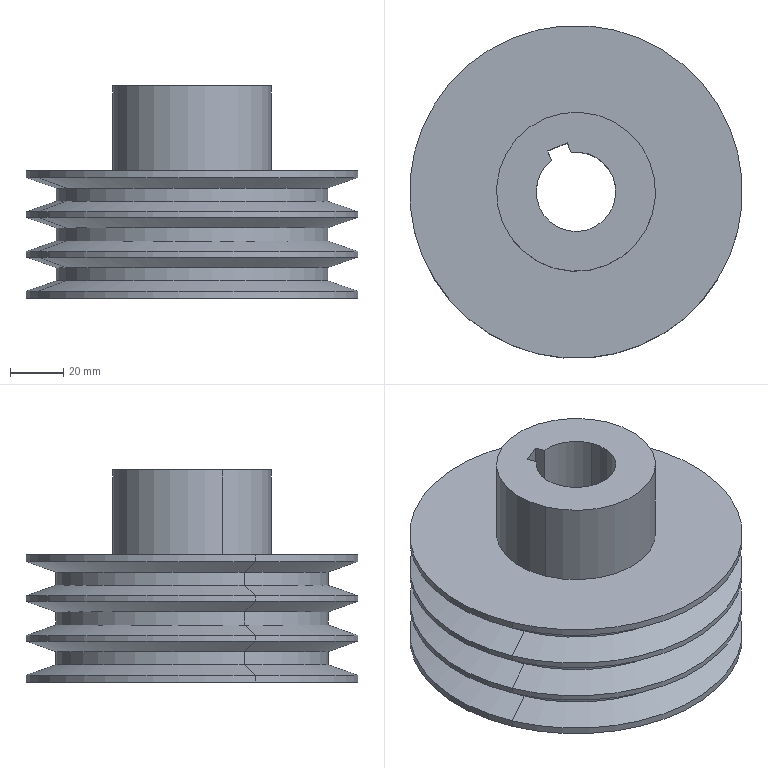Component | SolidWorks | SmallPulley-2 | 1 solid | 47 faces | box 125.5 x 125.5 x 80 mm | volume 513593 mm3 | cylinder 22 | cone 18 | plane 7 | commonest cylinder face diameters 125.5 x8 30 x6 102.6 x6 60 x2
build123d program:
from build123d import *

# Parameters (mm, degrees)
LPATTERN1_COUNT     = 3
LPATTERN1_PITCH     = 15
CHAMFER1_SIZE       = 1
SKETCH4_W           = 8
SKETCH4_H           = 3.843
CUT_EXTRUDE1_DEPTH  = 102.858
SKETCH5_R           = 30
BOSS_EXTRUDE1_DEPTH = 30


with BuildPart() as part:
    # Sketch1 → Revolve1 (revolve)
    with BuildSketch(Plane.XY, mode=Mode.PRIVATE) as revolve1_sk:
        Polygon((0, 15), (0, 62.75), (48, 62.75), (48, 30), (50, 30), (50, 15), align=None)
    revolve(revolve1_sk.sketch.rotate(Axis((0, 0, 0), (1, 0, 0)), 90), axis=Axis((0, 0, 0), (1, 0, 0)))

    # Sketch2 → Cut-Revolve1 (revolve, cut)
    with BuildSketch(Plane.XY, mode=Mode.PRIVATE) as cut_revolve1_sk:
        Polygon((11.504, 51.3), (15.447, 62.75), (2.553, 62.75), (6.496, 51.3), align=None)
    cut_revolve1 = revolve(cut_revolve1_sk.sketch.rotate(Axis((0, 0, 0), (1, 0, 0)), 90), axis=Axis((0, 0, 0), (1, 0, 0)), mode=Mode.SUBTRACT)

    # LPattern1: Cut-Revolve1 ×3
    with Locations(*[(i * LPATTERN1_PITCH, 0, 0) for i in range(1, LPATTERN1_COUNT)]):
        add(cut_revolve1, mode=Mode.SUBTRACT)

    # Chamfer1
    chamfer1_edges = [part.edges().sort_by_distance(p)[0] for p in [
        (50, 0, -15),
        (0, 0, -15),
    ]]
    chamfer(chamfer1_edges, length=CHAMFER1_SIZE)

    # Sketch4 → Cut-Extrude1 (cut, through all)
    with BuildSketch(Plane.ZY):
        with Locations((0, 16.378)):
            Rectangle(SKETCH4_W, SKETCH4_H)
    extrude(amount=-CUT_EXTRUDE1_DEPTH, mode=Mode.SUBTRACT)

    # Sketch5 → Boss-Extrude1 (add)
    with BuildSketch(Plane(origin=(50, 0, 0), x_dir=(0, 0, -1), z_dir=(1, 0, 0))):
        with Locations(Location((0, 0, 0), (0, 0, 180))):
            Circle(SKETCH5_R)
        with BuildLine():
            Line((-4, 14.457), (-4, 15.492))
            Line((-4, 15.492), (-4, 18.3))
            Line((-4, 18.3), (4, 18.3))
            Line((4, 18.3), (4, 15.492))
            Line((4, 15.492), (4, 14.457))
            ThreePointArc((4, 14.457), (0, -15), (-4, 14.457))
        make_face(mode=Mode.SUBTRACT)
    extrude(amount=BOSS_EXTRUDE1_DEPTH)


solid = part.part

# Placed as in the assembly
solid = solid.moved(Location((-814.935, 937.863, -11.2), (90, -67.477, 90)))